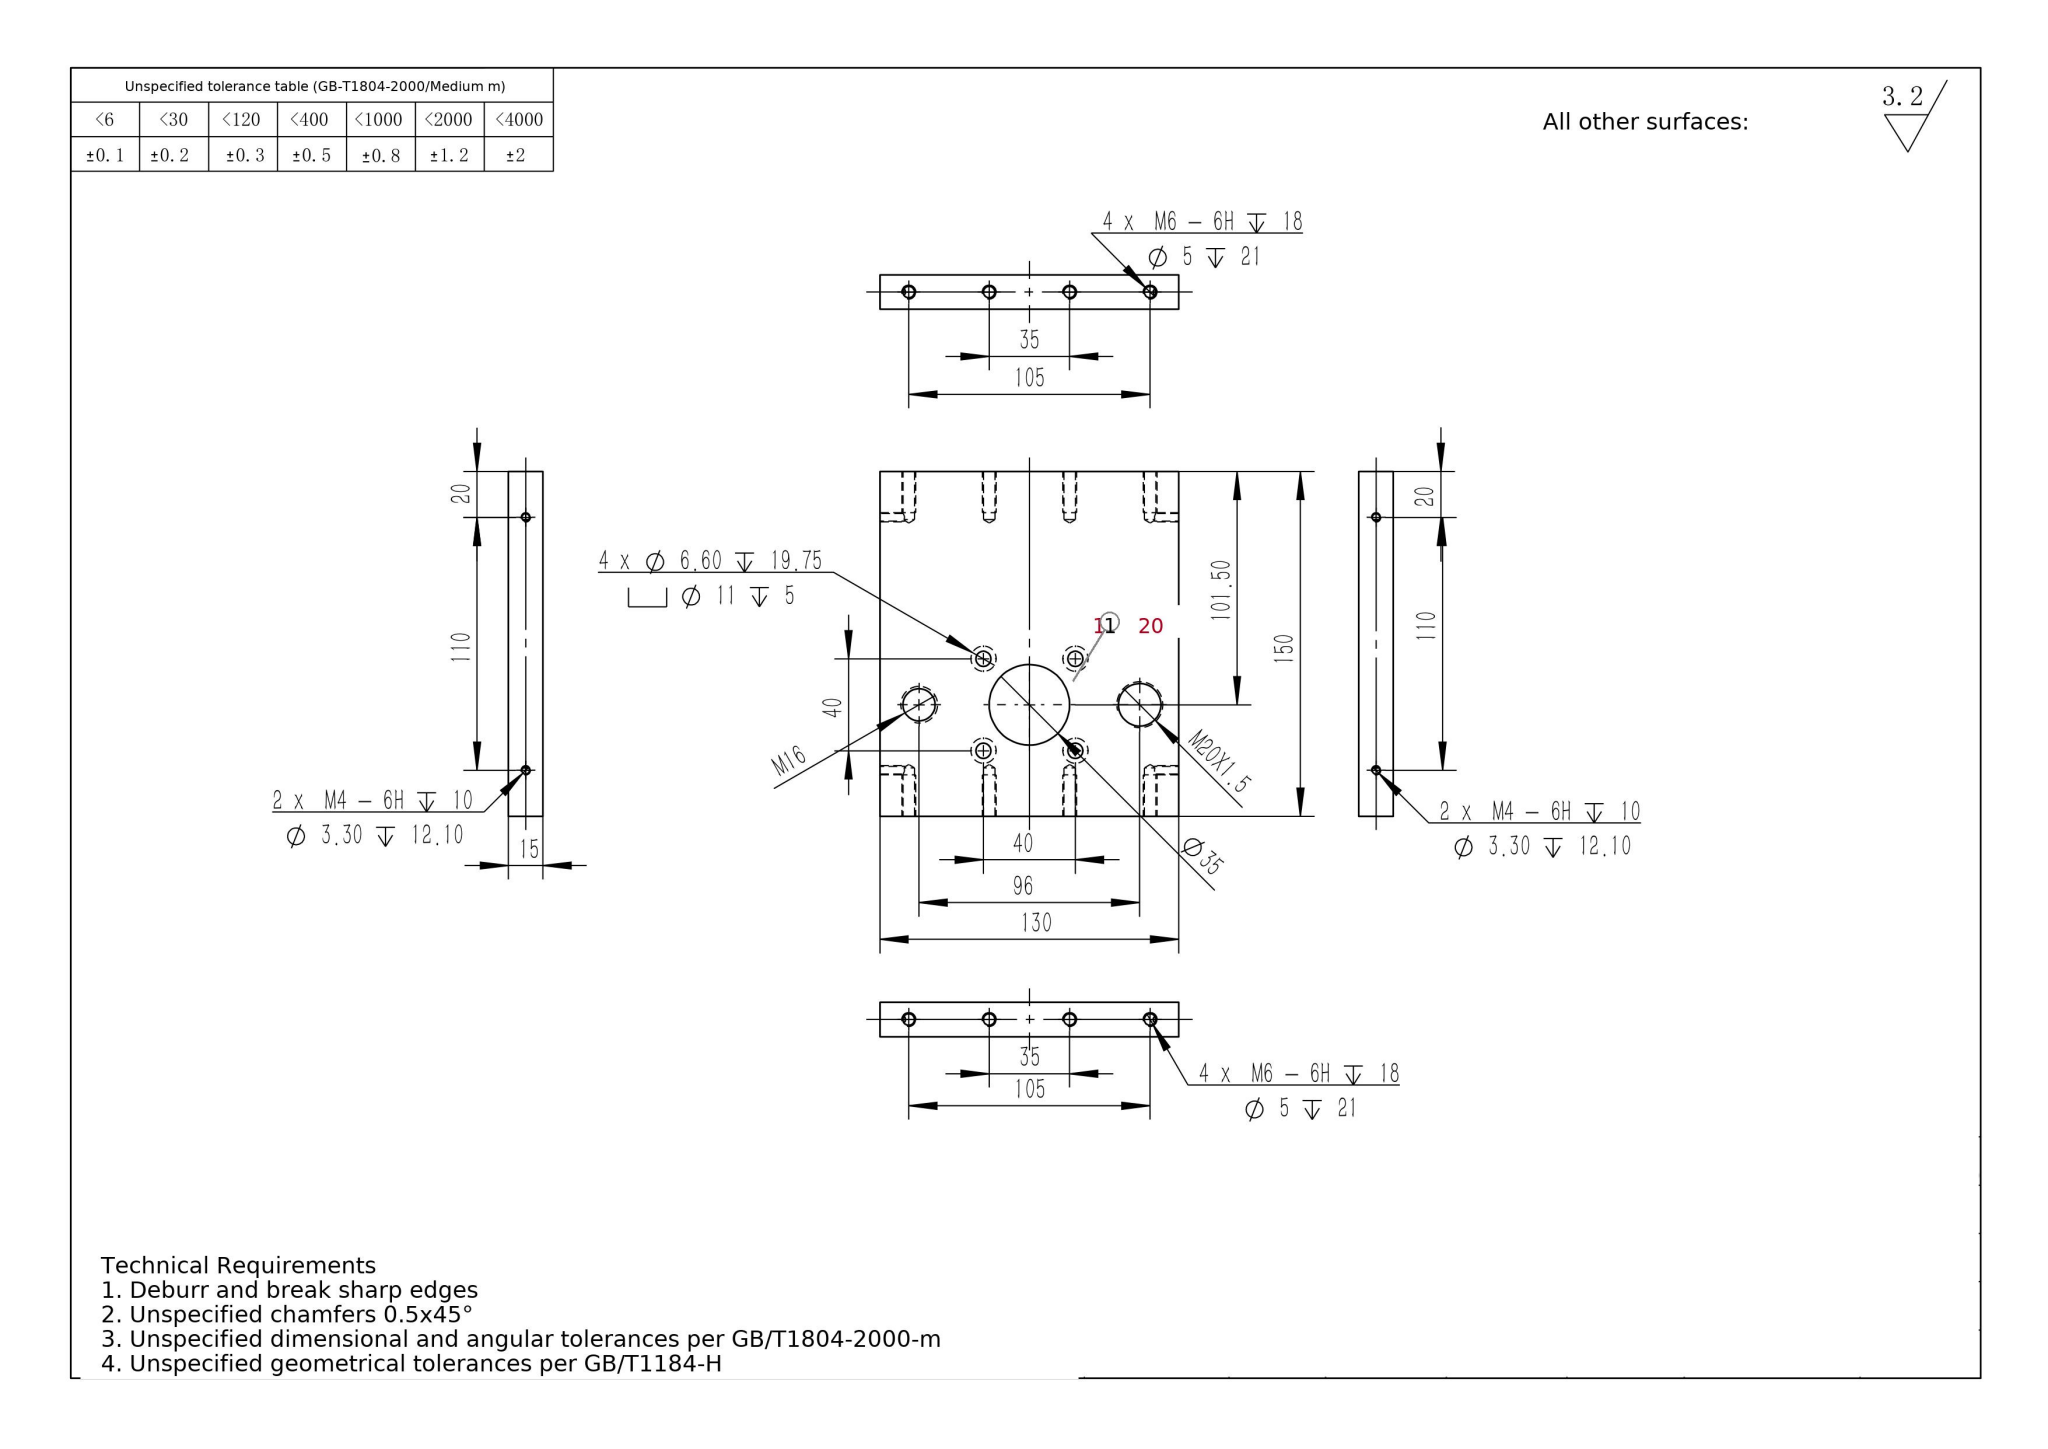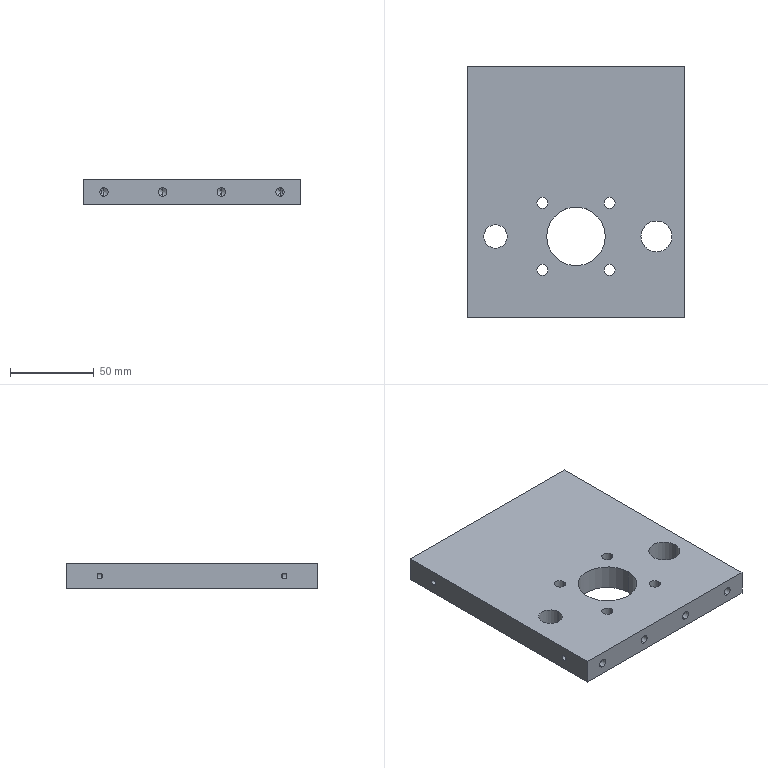Part | SolidWorks | mm | 1 solid | 72 faces | box 130 x 150 x 15 mm | volume 264731 mm3 | cylinder 46 | cone 16 | plane 10 | commonest cylinder face diameters 5 x16 3.3 x8 11 x8 6.6 x8 14 x2 18.5 x2 35 x2
build123d program:
from build123d import *

# Parameters (mm, degrees)
SKETCH1_W                                         = 130
SKETCH1_H                                         = 150
BOSS_EXTRUDE1_DEPTH                               = 15
SKETCH2_R                                         = 17.5
CUT_EXTRUDE1_DEPTH                                = 101.374
HOLE_SIZE_ACCORDING_TO_HEXAGON_SOCKET_D           = 6.6
HOLE_SIZE_ACCORDING_TO_HEXAGON_SOCKET_DEPTH       = 19.75
HOLE_SIZE_ACCORDING_TO_HEXAGON_SOCKET_CBORE_D     = 11
HOLE_SIZE_ACCORDING_TO_HEXAGON_SOCKET_CBORE_DEPTH = 5
HOLE_SIZE_ACCORDING_TO_HEXAGON_SOCKET_TIP         = 1.983
M6_TAPPED_HOLE1_AT_2_COUNT                        = 2
M6_TAPPED_HOLE1_AT_2_PITCH                        = 35
M6_TAPPED_HOLE1_AT_3_COUNT                        = 2
M6_TAPPED_HOLE1_AT_3_PITCH                        = 70
M6_TAPPED_HOLE1_AT_4_COUNT                        = 2
M6_TAPPED_HOLE1_AT_4_PITCH                        = 105
M20X1_5_TAPPED_HOLE1_D                            = 18.5
M20X1_5_TAPPED_HOLE1_DEPTH                        = 44.5
M20X1_5_TAPPED_HOLE1_TIP                          = 5.558
M16_TAPPED_HOLE1_D                                = 14
M16_TAPPED_HOLE1_DEPTH                            = 38
M16_TAPPED_HOLE1_TIP                              = 4.206
M4_TAPPED_HOLE1_AT_2_COUNT                        = 2
M4_TAPPED_HOLE1_AT_2_PITCH                        = 110


with BuildPart() as part:
    # Sketch1 → Boss-Extrude1 (new body)
    with BuildSketch(Plane.XY):
        Rectangle(SKETCH1_W, SKETCH1_H)
    extrude(amount=BOSS_EXTRUDE1_DEPTH)

    # Sketch2 → Cut-Extrude1 (cut, through all)
    with BuildSketch(Plane(origin=(0, 0, 0), x_dir=(-1, 0, 0), z_dir=(0, 0, -1))):
        with Locations((0, -26.5)):
            Circle(SKETCH2_R)
    extrude(amount=-CUT_EXTRUDE1_DEPTH, mode=Mode.SUBTRACT)

    # Hole Size _ according to_ Hexagon Socket
    with Locations(Plane(origin=(0, 0, 0), x_dir=(-1, 0, 0), z_dir=(0, 0, -1))):
        with Locations((20, -46.5), (-20, -6.5), (20, -6.5), (-20, -46.5)):
            CounterBoreHole(HOLE_SIZE_ACCORDING_TO_HEXAGON_SOCKET_D / 2, HOLE_SIZE_ACCORDING_TO_HEXAGON_SOCKET_CBORE_D / 2, HOLE_SIZE_ACCORDING_TO_HEXAGON_SOCKET_CBORE_DEPTH, depth=HOLE_SIZE_ACCORDING_TO_HEXAGON_SOCKET_DEPTH)
            with Locations((0, 0, -(HOLE_SIZE_ACCORDING_TO_HEXAGON_SOCKET_DEPTH + HOLE_SIZE_ACCORDING_TO_HEXAGON_SOCKET_TIP / 2))):  # 118° drill point
                Cone(0, HOLE_SIZE_ACCORDING_TO_HEXAGON_SOCKET_D / 2, HOLE_SIZE_ACCORDING_TO_HEXAGON_SOCKET_TIP, mode=Mode.SUBTRACT)

    # Sketch6 → M6 Tapped Hole1 (revolve, cut)
    with BuildSketch(Plane(origin=(-52.5, 75, 7.5), x_dir=(0, 0, 1), z_dir=(1, 0, 0))):
        Polygon((0, 0), (0, 22.502), (2.5, 21), (2.5, 0), align=None)
    m6_tapped_hole1 = revolve(axis=Axis((-52.5, 81.35, 7.5), (0, -1, 0)), mode=Mode.SUBTRACT)

    # M6 Tapped Hole1 at 2: M6 Tapped Hole1 ×2
    with Locations(*[(i * M6_TAPPED_HOLE1_AT_2_PITCH, 0, 0) for i in range(1, M6_TAPPED_HOLE1_AT_2_COUNT)]):
        add(m6_tapped_hole1, mode=Mode.SUBTRACT)

    # M6 Tapped Hole1 at 3: M6 Tapped Hole1 ×2
    with Locations(*[(i * M6_TAPPED_HOLE1_AT_3_PITCH, 0, 0) for i in range(1, M6_TAPPED_HOLE1_AT_3_COUNT)]):
        add(m6_tapped_hole1, mode=Mode.SUBTRACT)

    # M6 Tapped Hole1 at 4: M6 Tapped Hole1 ×2
    with Locations(*[(i * M6_TAPPED_HOLE1_AT_4_PITCH, 0, 0) for i in range(1, M6_TAPPED_HOLE1_AT_4_COUNT)]):
        add(m6_tapped_hole1, mode=Mode.SUBTRACT)

    # Mirror1: M6 Tapped Hole1 across plane
    add(m6_tapped_hole1.mirror(Plane.ZX), mode=Mode.SUBTRACT)

    # Mirror1 copy 1 sketch → Mirror1 copy 1 (revolve, cut)
    with BuildSketch(Plane(origin=(-17.5, -75, 7.5), x_dir=(0, 0, 1), z_dir=(1, 0, 0))):
        Polygon((0, 0), (0, -22.502), (2.5, -21), (2.5, 0), align=None)
    revolve(axis=Axis((-17.5, -81.35, 7.5), (0, -1, 0)), mode=Mode.SUBTRACT)

    # Mirror1 copy 2 sketch → Mirror1 copy 2 (revolve, cut)
    with BuildSketch(Plane(origin=(17.5, -75, 7.5), x_dir=(0, 0, 1), z_dir=(1, 0, 0))):
        Polygon((0, 0), (0, -22.502), (2.5, -21), (2.5, 0), align=None)
    revolve(axis=Axis((17.5, -81.35, 7.5), (0, -1, 0)), mode=Mode.SUBTRACT)

    # Mirror1 copy 3 sketch → Mirror1 copy 3 (revolve, cut)
    with BuildSketch(Plane(origin=(52.5, -75, 7.5), x_dir=(0, 0, 1), z_dir=(1, 0, 0))):
        Polygon((0, 0), (0, -22.502), (2.5, -21), (2.5, 0), align=None)
    revolve(axis=Axis((52.5, -81.35, 7.5), (0, -1, 0)), mode=Mode.SUBTRACT)

    # M20x1.5 Tapped Hole1
    with Locations(Plane(origin=(0, 0, 0), x_dir=(-1, 0, 0), z_dir=(0, 0, -1))):
        with Locations((-48, -26.5)):
            Hole(M20X1_5_TAPPED_HOLE1_D / 2, depth=M20X1_5_TAPPED_HOLE1_DEPTH)
            with Locations((0, 0, -(M20X1_5_TAPPED_HOLE1_DEPTH + M20X1_5_TAPPED_HOLE1_TIP / 2))):  # 118° drill point
                Cone(0, M20X1_5_TAPPED_HOLE1_D / 2, M20X1_5_TAPPED_HOLE1_TIP, mode=Mode.SUBTRACT)

    # M16 Tapped Hole1
    with Locations(Plane(origin=(0, 0, 0), x_dir=(-1, 0, 0), z_dir=(0, 0, -1))):
        with Locations((48, -26.5)):
            Hole(M16_TAPPED_HOLE1_D / 2, depth=M16_TAPPED_HOLE1_DEPTH)
            with Locations((0, 0, -(M16_TAPPED_HOLE1_DEPTH + M16_TAPPED_HOLE1_TIP / 2))):  # 118° drill point
                Cone(0, M16_TAPPED_HOLE1_D / 2, M16_TAPPED_HOLE1_TIP, mode=Mode.SUBTRACT)

    # Sketch12 → M4 Tapped Hole1 (revolve, cut)
    with BuildSketch(Plane(origin=(-65, 55, 7.5), x_dir=(0, 0, 1), z_dir=(0, 1, 0))):
        Polygon((0, 0), (0, 13.091), (1.65, 12.1), (1.65, 0), align=None)
    m4_tapped_hole1 = revolve(axis=Axis((-71.35, 55, 7.5), (1, 0, 0)), mode=Mode.SUBTRACT)

    # M4 Tapped Hole1 at 2: M4 Tapped Hole1 ×2
    with Locations(*[(0, -i * M4_TAPPED_HOLE1_AT_2_PITCH, 0) for i in range(1, M4_TAPPED_HOLE1_AT_2_COUNT)]):
        add(m4_tapped_hole1, mode=Mode.SUBTRACT)

    # Mirror2: M4 Tapped Hole1 across plane
    add(m4_tapped_hole1.mirror(Plane(origin=(0, 0, 0), x_dir=(0, 0, 1), z_dir=(1, 0, 0))), mode=Mode.SUBTRACT)

    # Mirror2 copy 1 sketch → Mirror2 copy 1 (revolve, cut)
    with BuildSketch(Plane(origin=(65, -55, 7.5), x_dir=(0, 0, 1), z_dir=(0, 1, 0))):
        Polygon((0, 0), (0, -13.091), (1.65, -12.1), (1.65, 0), align=None)
    revolve(axis=Axis((71.35, -55, 7.5), (1, 0, 0)), mode=Mode.SUBTRACT)


solid = part.part